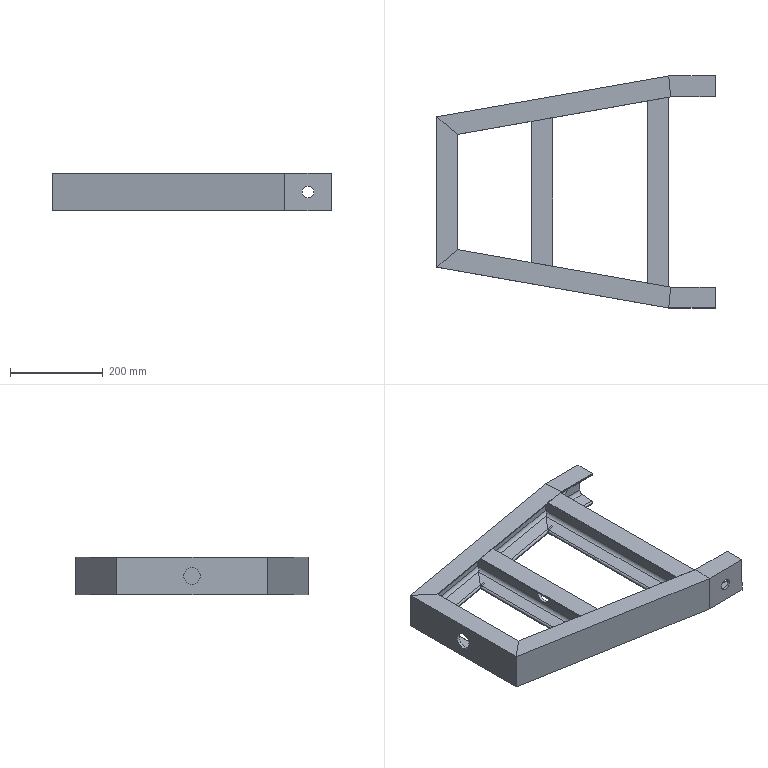Component | SolidWorks | 7TractionFrame-1 | 7 solids | 130 faces | volume 2363427 mm3 | plane 94 | cylinder 36 | commonest cylinder face diameters 8 x14 16 x14 25 x4 36 x4